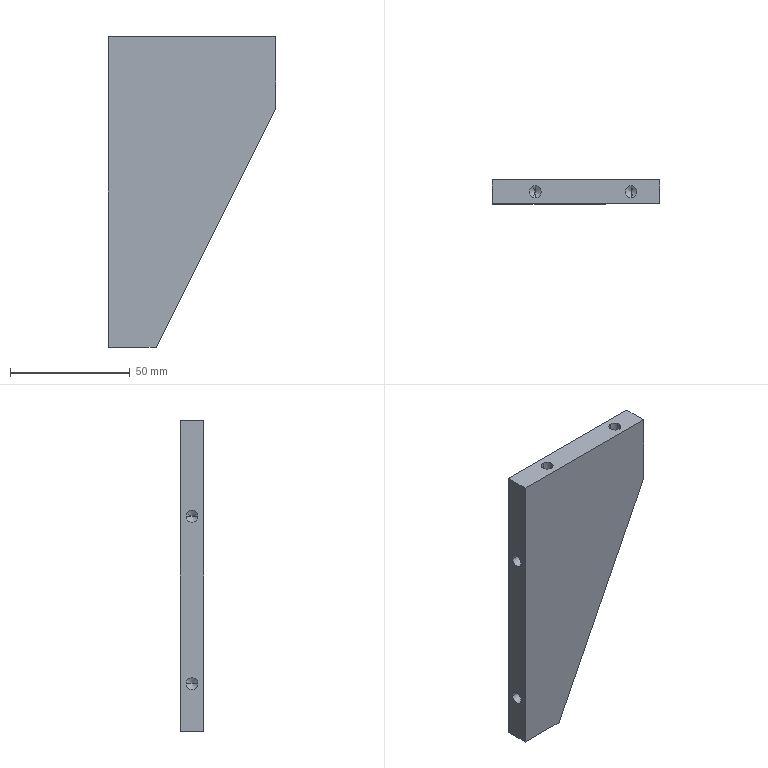Component | SolidWorks | 01-06MarkingMachineMountingReinforcementPlate-1 | 1 solid | 23 faces | box 70 x 10 x 130 mm | volume 64783 mm3 | cylinder 8 | cone 8 | plane 7 | commonest cylinder face diameters 5 x8 | material A3 Steel
build123d program:
from build123d import *

# Parameters (mm, degrees)
BOSS_EXTRUDE1_DEPTH   = 5
M6_TAPPED_HOLE1_D     = 5
M6_TAPPED_HOLE1_DEPTH = 15
M6_TAPPED_HOLE1_TIP   = 1.502
M6_TAPPED_HOLE2_D     = 5
M6_TAPPED_HOLE2_DEPTH = 15
M6_TAPPED_HOLE2_TIP   = 1.502


with BuildPart() as part:
    # Sketch1 → Boss-Extrude1 (new, symmetric)
    with BuildSketch(Plane.XY):
        Polygon((0, 130), (0, 0), (-70, 0), (-70, 30), (-20, 130), align=None)
    extrude(amount=BOSS_EXTRUDE1_DEPTH, both=True)

    # M6 Tapped Hole1
    with Locations(Plane(origin=(0, 110, 0), x_dir=(0, 0, 1), z_dir=(1, 0, 0))):
        with Locations((0, 0), (0, 70)):
            Hole(M6_TAPPED_HOLE1_D / 2, depth=M6_TAPPED_HOLE1_DEPTH)
            with Locations((0, 0, -(M6_TAPPED_HOLE1_DEPTH + M6_TAPPED_HOLE1_TIP / 2))):  # 118° drill point
                Cone(0, M6_TAPPED_HOLE1_D / 2, M6_TAPPED_HOLE1_TIP, mode=Mode.SUBTRACT)

    # M6 Tapped Hole2
    with Locations(Plane(origin=(-18, 0, 0), x_dir=(-1, 0, 0), z_dir=(0, -1, 0))):
        with Locations((0, 0), (40, 0)):
            Hole(M6_TAPPED_HOLE2_D / 2, depth=M6_TAPPED_HOLE2_DEPTH)
            with Locations((0, 0, -(M6_TAPPED_HOLE2_DEPTH + M6_TAPPED_HOLE2_TIP / 2))):  # 118° drill point
                Cone(0, M6_TAPPED_HOLE2_D / 2, M6_TAPPED_HOLE2_TIP, mode=Mode.SUBTRACT)


solid = part.part

# Placed as in the assembly
solid = solid.moved(Location((-46.91, 2.41, 85), (90, 0, -180)))
STEP:
#1=CARTESIAN_POINT('',(-1.138,-0.003525,2.756));
#2=VERTEX_POINT('',#1);
#3=CARTESIAN_POINT('',(-1.138,0.1933,2.756));
#4=VERTEX_POINT('',#3);
#5=CARTESIAN_POINT('',(-1.138,0.0949,2.756));
#6=DIRECTION('',(0.,0.,1.));
#7=DIRECTION('',(0.,1.,0.));
#8=AXIS2_PLACEMENT_3D('',#5,#6,#7);
#9=CIRCLE('',#8,0.09843);
#10=EDGE_CURVE('',#2,#4,#9,.T.);
#11=ORIENTED_EDGE('',*,*,#10,.F.);
#12=CARTESIAN_POINT('',(-1.138,-0.003525,3.346));
#13=VERTEX_POINT('',#12);
#14=CARTESIAN_POINT('',(-1.138,-0.003525,3.346));
#15=DIRECTION('',(0.,0.,1.));
#16=VECTOR('',#15,39.37);
#17=LINE('',#14,#16);
#18=EDGE_CURVE('',#2,#13,#17,.T.);
#19=ORIENTED_EDGE('',*,*,#18,.T.);
#20=CARTESIAN_POINT('',(-1.138,0.1933,3.346));
#21=VERTEX_POINT('',#20);
#22=CARTESIAN_POINT('',(-1.138,0.0949,3.346));
#23=DIRECTION('',(0.,0.,1.));
#24=DIRECTION('',(0.,1.,0.));
#25=AXIS2_PLACEMENT_3D('',#22,#23,#24);
#26=CIRCLE('',#25,0.09843);
#27=EDGE_CURVE('',#13,#21,#26,.T.);
#28=ORIENTED_EDGE('',*,*,#27,.T.);
#29=CARTESIAN_POINT('',(-1.138,0.1933,3.346));
#30=DIRECTION('',(0.,0.,1.));
#31=VECTOR('',#30,39.37);
#32=LINE('',#29,#31);
#33=EDGE_CURVE('',#4,#21,#32,.T.);
#34=ORIENTED_EDGE('',*,*,#33,.F.);
#35=EDGE_LOOP('',(#11,#19,#28,#34));
#36=FACE_OUTER_BOUND('',#35,.T.);
#37=CARTESIAN_POINT('',(-1.138,0.0949,3.346));
#38=DIRECTION('',(0.,0.,1.));
#39=DIRECTION('',(0.,1.,0.));
#40=AXIS2_PLACEMENT_3D('',#37,#38,#39);
#41=CYLINDRICAL_SURFACE('',#40,0.09843);
#42=ADVANCED_FACE('',(#36),#41,.F.);
#43=CARTESIAN_POINT('',(-1.138,0.0949,2.697));
#44=VERTEX_POINT('',#43);
#45=CARTESIAN_POINT('',(-1.138,0.1933,2.756));
#46=DIRECTION('',(0.,0.8572,0.515));
#47=VECTOR('',#46,39.37);
#48=LINE('',#45,#47);
#49=EDGE_CURVE('',#44,#4,#48,.T.);
#50=ORIENTED_EDGE('',*,*,#49,.F.);
#51=CARTESIAN_POINT('',(-1.138,-0.003525,2.756));
#52=DIRECTION('',(0.,-0.8572,0.515));
#53=VECTOR('',#52,39.37);
#54=LINE('',#51,#53);
#55=EDGE_CURVE('',#44,#2,#54,.T.);
#56=ORIENTED_EDGE('',*,*,#55,.T.);
#57=ORIENTED_EDGE('',*,*,#10,.T.);
#58=EDGE_LOOP('',(#50,#56,#57));
#59=FACE_OUTER_BOUND('',#58,.T.);
#60=CARTESIAN_POINT('',(-1.138,0.0949,2.756));
#61=DIRECTION('',(0.,0.,1.));
#62=DIRECTION('',(0.,1.,0.));
#63=AXIS2_PLACEMENT_3D('',#60,#61,#62);
#64=CONICAL_SURFACE('',#63,0.09843,1.03);
#65=ADVANCED_FACE('',(#59),#64,.F.);
#66=CARTESIAN_POINT('',(0.4366,-0.003525,2.756));
#67=VERTEX_POINT('',#66);
#68=CARTESIAN_POINT('',(0.4366,0.1933,2.756));
#69=VERTEX_POINT('',#68);
#70=CARTESIAN_POINT('',(0.4366,0.0949,2.756));
#71=DIRECTION('',(0.,0.,1.));
#72=DIRECTION('',(0.,1.,0.));
#73=AXIS2_PLACEMENT_3D('',#70,#71,#72);
#74=CIRCLE('',#73,0.09843);
#75=EDGE_CURVE('',#67,#69,#74,.T.);
#76=ORIENTED_EDGE('',*,*,#75,.F.);
#77=CARTESIAN_POINT('',(0.4366,-0.003525,3.346));
#78=VERTEX_POINT('',#77);
#79=CARTESIAN_POINT('',(0.4366,-0.003525,3.346));
#80=DIRECTION('',(0.,0.,1.));
#81=VECTOR('',#80,39.37);
#82=LINE('',#79,#81);
#83=EDGE_CURVE('',#67,#78,#82,.T.);
#84=ORIENTED_EDGE('',*,*,#83,.T.);
#85=CARTESIAN_POINT('',(0.4366,0.1933,3.346));
#86=VERTEX_POINT('',#85);
#87=CARTESIAN_POINT('',(0.4366,0.0949,3.346));
#88=DIRECTION('',(0.,0.,1.));
#89=DIRECTION('',(0.,1.,0.));
#90=AXIS2_PLACEMENT_3D('',#87,#88,#89);
#91=CIRCLE('',#90,0.09843);
#92=EDGE_CURVE('',#78,#86,#91,.T.);
#93=ORIENTED_EDGE('',*,*,#92,.T.);
#94=CARTESIAN_POINT('',(0.4366,0.1933,3.346));
#95=DIRECTION('',(0.,0.,1.));
#96=VECTOR('',#95,39.37);
#97=LINE('',#94,#96);
#98=EDGE_CURVE('',#69,#86,#97,.T.);
#99=ORIENTED_EDGE('',*,*,#98,.F.);
#100=EDGE_LOOP('',(#76,#84,#93,#99));
#101=FACE_OUTER_BOUND('',#100,.T.);
#102=CARTESIAN_POINT('',(0.4366,0.0949,3.346));
#103=DIRECTION('',(0.,0.,1.));
#104=DIRECTION('',(0.,1.,0.));
#105=AXIS2_PLACEMENT_3D('',#102,#103,#104);
#106=CYLINDRICAL_SURFACE('',#105,0.09843);
#107=ADVANCED_FACE('',(#101),#106,.F.);
#108=CARTESIAN_POINT('',(0.4366,0.0949,2.697));
#109=VERTEX_POINT('',#108);
#110=CARTESIAN_POINT('',(0.4366,0.1933,2.756));
#111=DIRECTION('',(0.,0.8572,0.515));
#112=VECTOR('',#111,39.37);
#113=LINE('',#110,#112);
#114=EDGE_CURVE('',#109,#69,#113,.T.);
#115=ORIENTED_EDGE('',*,*,#114,.F.);
#116=CARTESIAN_POINT('',(0.4366,-0.003525,2.756));
#117=DIRECTION('',(0.,-0.8572,0.515));
#118=VECTOR('',#117,39.37);
#119=LINE('',#116,#118);
#120=EDGE_CURVE('',#109,#67,#119,.T.);
#121=ORIENTED_EDGE('',*,*,#120,.T.);
#122=ORIENTED_EDGE('',*,*,#75,.T.);
#123=EDGE_LOOP('',(#115,#121,#122));
#124=FACE_OUTER_BOUND('',#123,.T.);
#125=CARTESIAN_POINT('',(0.4366,0.0949,2.756));
#126=DIRECTION('',(0.,0.,1.));
#127=DIRECTION('',(0.,1.,0.));
#128=AXIS2_PLACEMENT_3D('',#125,#126,#127);
#129=CONICAL_SURFACE('',#128,0.09843,1.03);
#130=ADVANCED_FACE('',(#124),#129,.F.);
#131=CARTESIAN_POINT('',(-1.256,-0.003525,-0.9843));
#132=VERTEX_POINT('',#131);
#133=CARTESIAN_POINT('',(-1.256,0.1933,-0.9843));
#134=VERTEX_POINT('',#133);
#135=CARTESIAN_POINT('',(-1.256,0.0949,-0.9843));
#136=DIRECTION('',(-1.,-0.,0.));
#137=DIRECTION('',(0.,1.,0.));
#138=AXIS2_PLACEMENT_3D('',#135,#136,#137);
#139=CIRCLE('',#138,0.09843);
#140=EDGE_CURVE('',#132,#134,#139,.T.);
#141=ORIENTED_EDGE('',*,*,#140,.F.);
#142=CARTESIAN_POINT('',(-1.847,-0.003525,-0.9843));
#143=VERTEX_POINT('',#142);
#144=CARTESIAN_POINT('',(-1.847,-0.003525,-0.9843));
#145=DIRECTION('',(-1.,-0.,0.));
#146=VECTOR('',#145,39.37);
#147=LINE('',#144,#146);
#148=EDGE_CURVE('',#132,#143,#147,.T.);
#149=ORIENTED_EDGE('',*,*,#148,.T.);
#150=CARTESIAN_POINT('',(-1.847,0.1933,-0.9843));
#151=VERTEX_POINT('',#150);
#152=CARTESIAN_POINT('',(-1.847,0.0949,-0.9843));
#153=DIRECTION('',(-1.,-0.,0.));
#154=DIRECTION('',(0.,1.,0.));
#155=AXIS2_PLACEMENT_3D('',#152,#153,#154);
#156=CIRCLE('',#155,0.09843);
#157=EDGE_CURVE('',#143,#151,#156,.T.);
#158=ORIENTED_EDGE('',*,*,#157,.T.);
#159=CARTESIAN_POINT('',(-1.847,0.1933,-0.9843));
#160=DIRECTION('',(-1.,-0.,0.));
#161=VECTOR('',#160,39.37);
#162=LINE('',#159,#161);
#163=EDGE_CURVE('',#134,#151,#162,.T.);
#164=ORIENTED_EDGE('',*,*,#163,.F.);
#165=EDGE_LOOP('',(#141,#149,#158,#164));
#166=FACE_OUTER_BOUND('',#165,.T.);
#167=CARTESIAN_POINT('',(-1.847,0.0949,-0.9843));
#168=DIRECTION('',(-1.,-0.,0.));
#169=DIRECTION('',(0.,1.,0.));
#170=AXIS2_PLACEMENT_3D('',#167,#168,#169);
#171=CYLINDRICAL_SURFACE('',#170,0.09843);
#172=ADVANCED_FACE('',(#166),#171,.F.);
#173=CARTESIAN_POINT('',(-1.197,0.0949,-0.9843));
#174=VERTEX_POINT('',#173);
#175=CARTESIAN_POINT('',(-1.256,0.1933,-0.9843));
#176=DIRECTION('',(-0.515,0.8572,0.));
#177=VECTOR('',#176,39.37);
#178=LINE('',#175,#177);
#179=EDGE_CURVE('',#174,#134,#178,.T.);
#180=ORIENTED_EDGE('',*,*,#179,.F.);
#181=CARTESIAN_POINT('',(-1.256,-0.003525,-0.9843));
#182=DIRECTION('',(-0.515,-0.8572,0.));
#183=VECTOR('',#182,39.37);
#184=LINE('',#181,#183);
#185=EDGE_CURVE('',#174,#132,#184,.T.);
#186=ORIENTED_EDGE('',*,*,#185,.T.);
#187=ORIENTED_EDGE('',*,*,#140,.T.);
#188=EDGE_LOOP('',(#180,#186,#187));
#189=FACE_OUTER_BOUND('',#188,.T.);
#190=CARTESIAN_POINT('',(-1.256,0.0949,-0.9843));
#191=DIRECTION('',(-1.,-0.,0.));
#192=DIRECTION('',(0.,1.,0.));
#193=AXIS2_PLACEMENT_3D('',#190,#191,#192);
#194=CONICAL_SURFACE('',#193,0.09843,1.03);
#195=ADVANCED_FACE('',(#189),#194,.F.);
#196=CARTESIAN_POINT('',(-1.256,-0.003525,1.772));
#197=VERTEX_POINT('',#196);
#198=CARTESIAN_POINT('',(-1.256,0.1933,1.772));
#199=VERTEX_POINT('',#198);
#200=CARTESIAN_POINT('',(-1.256,0.0949,1.772));
#201=DIRECTION('',(-1.,-0.,0.));
#202=DIRECTION('',(0.,1.,0.));
#203=AXIS2_PLACEMENT_3D('',#200,#201,#202);
#204=CIRCLE('',#203,0.09843);
#205=EDGE_CURVE('',#197,#199,#204,.T.);
#206=ORIENTED_EDGE('',*,*,#205,.F.);
#207=CARTESIAN_POINT('',(-1.847,-0.003525,1.772));
#208=VERTEX_POINT('',#207);
#209=CARTESIAN_POINT('',(-1.847,-0.003525,1.772));
#210=DIRECTION('',(-1.,-0.,0.));
#211=VECTOR('',#210,39.37);
#212=LINE('',#209,#211);
#213=EDGE_CURVE('',#197,#208,#212,.T.);
#214=ORIENTED_EDGE('',*,*,#213,.T.);
#215=CARTESIAN_POINT('',(-1.847,0.1933,1.772));
#216=VERTEX_POINT('',#215);
#217=CARTESIAN_POINT('',(-1.847,0.0949,1.772));
#218=DIRECTION('',(-1.,-0.,0.));
#219=DIRECTION('',(0.,1.,0.));
#220=AXIS2_PLACEMENT_3D('',#217,#218,#219);
#221=CIRCLE('',#220,0.09843);
#222=EDGE_CURVE('',#208,#216,#221,.T.);
#223=ORIENTED_EDGE('',*,*,#222,.T.);
#224=CARTESIAN_POINT('',(-1.847,0.1933,1.772));
#225=DIRECTION('',(-1.,-0.,0.));
#226=VECTOR('',#225,39.37);
#227=LINE('',#224,#226);
#228=EDGE_CURVE('',#199,#216,#227,.T.);
#229=ORIENTED_EDGE('',*,*,#228,.F.);
#230=EDGE_LOOP('',(#206,#214,#223,#229));
#231=FACE_OUTER_BOUND('',#230,.T.);
#232=CARTESIAN_POINT('',(-1.847,0.0949,1.772));
#233=DIRECTION('',(-1.,-0.,0.));
#234=DIRECTION('',(0.,1.,0.));
#235=AXIS2_PLACEMENT_3D('',#232,#233,#234);
#236=CYLINDRICAL_SURFACE('',#235,0.09843);
#237=ADVANCED_FACE('',(#231),#236,.F.);
#238=CARTESIAN_POINT('',(-1.197,0.0949,1.772));
#239=VERTEX_POINT('',#238);
#240=CARTESIAN_POINT('',(-1.256,0.1933,1.772));
#241=DIRECTION('',(-0.515,0.8572,0.));
#242=VECTOR('',#241,39.37);
#243=LINE('',#240,#242);
#244=EDGE_CURVE('',#239,#199,#243,.T.);
#245=ORIENTED_EDGE('',*,*,#244,.F.);
#246=CARTESIAN_POINT('',(-1.256,-0.003525,1.772));
#247=DIRECTION('',(-0.515,-0.8572,0.));
#248=VECTOR('',#247,39.37);
#249=LINE('',#246,#248);
#250=EDGE_CURVE('',#239,#197,#249,.T.);
#251=ORIENTED_EDGE('',*,*,#250,.T.);
#252=ORIENTED_EDGE('',*,*,#205,.T.);
#253=EDGE_LOOP('',(#245,#251,#252));
#254=FACE_OUTER_BOUND('',#253,.T.);
#255=CARTESIAN_POINT('',(-1.256,0.0949,1.772));
#256=DIRECTION('',(-1.,-0.,0.));
#257=DIRECTION('',(0.,1.,0.));
#258=AXIS2_PLACEMENT_3D('',#255,#256,#257);
#259=CONICAL_SURFACE('',#258,0.09843,1.03);
#260=ADVANCED_FACE('',(#254),#259,.F.);
#261=CARTESIAN_POINT('',(-1.847,0.2918,-1.772));
#262=VERTEX_POINT('',#261);
#263=CARTESIAN_POINT('',(-1.059,0.2918,-1.772));
#264=VERTEX_POINT('',#263);
#265=CARTESIAN_POINT('',(-1.059,0.2918,-1.772));
#266=DIRECTION('',(1.,0.,-0.));
#267=VECTOR('',#266,39.37);
#268=LINE('',#265,#267);
#269=EDGE_CURVE('',#262,#264,#268,.T.);
#270=ORIENTED_EDGE('',*,*,#269,.T.);
#271=CARTESIAN_POINT('',(-1.059,-0.102,-1.772));
#272=VERTEX_POINT('',#271);
#273=CARTESIAN_POINT('',(-1.059,-0.102,-1.772));
#274=DIRECTION('',(-0.,1.,0.));
#275=VECTOR('',#274,39.37);
#276=LINE('',#273,#275);
#277=EDGE_CURVE('',#272,#264,#276,.T.);
#278=ORIENTED_EDGE('',*,*,#277,.F.);
#279=CARTESIAN_POINT('',(-1.847,-0.102,-1.772));
#280=VERTEX_POINT('',#279);
#281=CARTESIAN_POINT('',(-1.059,-0.102,-1.772));
#282=DIRECTION('',(1.,0.,-0.));
#283=VECTOR('',#282,39.37);
#284=LINE('',#281,#283);
#285=EDGE_CURVE('',#280,#272,#284,.T.);
#286=ORIENTED_EDGE('',*,*,#285,.F.);
#287=CARTESIAN_POINT('',(-1.847,-0.102,-1.772));
#288=DIRECTION('',(-0.,1.,0.));
#289=VECTOR('',#288,39.37);
#290=LINE('',#287,#289);
#291=EDGE_CURVE('',#280,#262,#290,.T.);
#292=ORIENTED_EDGE('',*,*,#291,.T.);
#293=EDGE_LOOP('',(#270,#278,#286,#292));
#294=FACE_OUTER_BOUND('',#293,.T.);
#295=CARTESIAN_POINT('',(-1.059,-0.102,-1.772));
#296=DIRECTION('',(0.,-0.,1.));
#297=DIRECTION('',(-0.,1.,0.));
#298=AXIS2_PLACEMENT_3D('',#295,#296,#297);
#299=PLANE('',#298);
#300=ADVANCED_FACE('',(#294),#299,.F.);
#301=CARTESIAN_POINT('',(0.909,0.2918,2.165));
#302=VERTEX_POINT('',#301);
#303=CARTESIAN_POINT('',(0.909,0.2918,2.165));
#304=DIRECTION('',(0.4472,0.,0.8944));
#305=VECTOR('',#304,39.37);
#306=LINE('',#303,#305);
#307=EDGE_CURVE('',#264,#302,#306,.T.);
#308=ORIENTED_EDGE('',*,*,#307,.T.);
#309=CARTESIAN_POINT('',(0.909,-0.102,2.165));
#310=VERTEX_POINT('',#309);
#311=CARTESIAN_POINT('',(0.909,-0.102,2.165));
#312=DIRECTION('',(-0.,1.,0.));
#313=VECTOR('',#312,39.37);
#314=LINE('',#311,#313);
#315=EDGE_CURVE('',#310,#302,#314,.T.);
#316=ORIENTED_EDGE('',*,*,#315,.F.);
#317=CARTESIAN_POINT('',(0.909,-0.102,2.165));
#318=DIRECTION('',(0.4472,0.,0.8944));
#319=VECTOR('',#318,39.37);
#320=LINE('',#317,#319);
#321=EDGE_CURVE('',#272,#310,#320,.T.);
#322=ORIENTED_EDGE('',*,*,#321,.F.);
#323=ORIENTED_EDGE('',*,*,#277,.T.);
#324=EDGE_LOOP('',(#308,#316,#322,#323));
#325=FACE_OUTER_BOUND('',#324,.T.);
#326=CARTESIAN_POINT('',(0.909,-0.102,2.165));
#327=DIRECTION('',(-0.8944,-0.,0.4472));
#328=DIRECTION('',(-0.4472,-0.,-0.8944));
#329=AXIS2_PLACEMENT_3D('',#326,#327,#328);
#330=PLANE('',#329);
#331=ADVANCED_FACE('',(#325),#330,.F.);
#332=CARTESIAN_POINT('',(0.909,0.2918,3.346));
#333=VERTEX_POINT('',#332);
#334=CARTESIAN_POINT('',(0.909,0.2918,3.346));
#335=DIRECTION('',(0.,0.,1.));
#336=VECTOR('',#335,39.37);
#337=LINE('',#334,#336);
#338=EDGE_CURVE('',#302,#333,#337,.T.);
#339=ORIENTED_EDGE('',*,*,#338,.T.);
#340=CARTESIAN_POINT('',(0.909,-0.102,3.346));
#341=VERTEX_POINT('',#340);
#342=CARTESIAN_POINT('',(0.909,-0.102,3.346));
#343=DIRECTION('',(-0.,1.,0.));
#344=VECTOR('',#343,39.37);
#345=LINE('',#342,#344);
#346=EDGE_CURVE('',#341,#333,#345,.T.);
#347=ORIENTED_EDGE('',*,*,#346,.F.);
#348=CARTESIAN_POINT('',(0.909,-0.102,3.346));
#349=DIRECTION('',(0.,0.,1.));
#350=VECTOR('',#349,39.37);
#351=LINE('',#348,#350);
#352=EDGE_CURVE('',#310,#341,#351,.T.);
#353=ORIENTED_EDGE('',*,*,#352,.F.);
#354=ORIENTED_EDGE('',*,*,#315,.T.);
#355=EDGE_LOOP('',(#339,#347,#353,#354));
#356=FACE_OUTER_BOUND('',#355,.T.);
#357=CARTESIAN_POINT('',(0.909,-0.102,3.346));
#358=DIRECTION('',(-1.,-0.,0.));
#359=DIRECTION('',(-0.,1.,0.));
#360=AXIS2_PLACEMENT_3D('',#357,#358,#359);
#361=PLANE('',#360);
#362=ADVANCED_FACE('',(#356),#361,.F.);
#363=CARTESIAN_POINT('',(-1.138,0.0949,3.346));
#364=DIRECTION('',(0.,0.,1.));
#365=DIRECTION('',(0.,1.,0.));
#366=AXIS2_PLACEMENT_3D('',#363,#364,#365);
#367=CIRCLE('',#366,0.09843);
#368=EDGE_CURVE('',#21,#13,#367,.T.);
#369=ORIENTED_EDGE('',*,*,#368,.F.);
#370=ORIENTED_EDGE('',*,*,#27,.F.);
#371=EDGE_LOOP('',(#369,#370));
#372=FACE_BOUND('',#371,.T.);
#373=CARTESIAN_POINT('',(0.4366,0.0949,3.346));
#374=DIRECTION('',(0.,0.,1.));
#375=DIRECTION('',(0.,1.,0.));
#376=AXIS2_PLACEMENT_3D('',#373,#374,#375);
#377=CIRCLE('',#376,0.09843);
#378=EDGE_CURVE('',#86,#78,#377,.T.);
#379=ORIENTED_EDGE('',*,*,#378,.F.);
#380=ORIENTED_EDGE('',*,*,#92,.F.);
#381=EDGE_LOOP('',(#379,#380));
#382=FACE_BOUND('',#381,.T.);
#383=CARTESIAN_POINT('',(-1.847,0.2918,3.346));
#384=VERTEX_POINT('',#383);
#385=CARTESIAN_POINT('',(-1.847,0.2918,3.346));
#386=DIRECTION('',(-1.,-0.,0.));
#387=VECTOR('',#386,39.37);
#388=LINE('',#385,#387);
#389=EDGE_CURVE('',#333,#384,#388,.T.);
#390=ORIENTED_EDGE('',*,*,#389,.T.);
#391=CARTESIAN_POINT('',(-1.847,-0.102,3.346));
#392=VERTEX_POINT('',#391);
#393=CARTESIAN_POINT('',(-1.847,-0.102,3.346));
#394=DIRECTION('',(-0.,1.,0.));
#395=VECTOR('',#394,39.37);
#396=LINE('',#393,#395);
#397=EDGE_CURVE('',#392,#384,#396,.T.);
#398=ORIENTED_EDGE('',*,*,#397,.F.);
#399=CARTESIAN_POINT('',(-1.847,-0.102,3.346));
#400=DIRECTION('',(-1.,-0.,0.));
#401=VECTOR('',#400,39.37);
#402=LINE('',#399,#401);
#403=EDGE_CURVE('',#341,#392,#402,.T.);
#404=ORIENTED_EDGE('',*,*,#403,.F.);
#405=ORIENTED_EDGE('',*,*,#346,.T.);
#406=EDGE_LOOP('',(#390,#398,#404,#405));
#407=FACE_OUTER_BOUND('',#406,.T.);
#408=CARTESIAN_POINT('',(-1.847,-0.102,3.346));
#409=DIRECTION('',(-0.,0.,-1.));
#410=DIRECTION('',(1.,0.,-0.));
#411=AXIS2_PLACEMENT_3D('',#408,#409,#410);
#412=PLANE('',#411);
#413=ADVANCED_FACE('',(#372,#382,#407),#412,.F.);
#414=CARTESIAN_POINT('',(-1.847,0.0949,-0.9843));
#415=DIRECTION('',(-1.,-0.,0.));
#416=DIRECTION('',(0.,1.,0.));
#417=AXIS2_PLACEMENT_3D('',#414,#415,#416);
#418=CIRCLE('',#417,0.09843);
#419=EDGE_CURVE('',#151,#143,#418,.T.);
#420=ORIENTED_EDGE('',*,*,#419,.F.);
#421=ORIENTED_EDGE('',*,*,#157,.F.);
#422=EDGE_LOOP('',(#420,#421));
#423=FACE_BOUND('',#422,.T.);
#424=CARTESIAN_POINT('',(-1.847,0.0949,1.772));
#425=DIRECTION('',(-1.,-0.,0.));
#426=DIRECTION('',(0.,1.,0.));
#427=AXIS2_PLACEMENT_3D('',#424,#425,#426);
#428=CIRCLE('',#427,0.09843);
#429=EDGE_CURVE('',#216,#208,#428,.T.);
#430=ORIENTED_EDGE('',*,*,#429,.F.);
#431=ORIENTED_EDGE('',*,*,#222,.F.);
#432=EDGE_LOOP('',(#430,#431));
#433=FACE_BOUND('',#432,.T.);
#434=CARTESIAN_POINT('',(-1.847,0.2918,-1.772));
#435=DIRECTION('',(-0.,-0.,-1.));
#436=VECTOR('',#435,39.37);
#437=LINE('',#434,#436);
#438=EDGE_CURVE('',#384,#262,#437,.T.);
#439=ORIENTED_EDGE('',*,*,#438,.T.);
#440=ORIENTED_EDGE('',*,*,#291,.F.);
#441=CARTESIAN_POINT('',(-1.847,-0.102,-1.772));
#442=DIRECTION('',(-0.,-0.,-1.));
#443=VECTOR('',#442,39.37);
#444=LINE('',#441,#443);
#445=EDGE_CURVE('',#392,#280,#444,.T.);
#446=ORIENTED_EDGE('',*,*,#445,.F.);
#447=ORIENTED_EDGE('',*,*,#397,.T.);
#448=EDGE_LOOP('',(#439,#440,#446,#447));
#449=FACE_OUTER_BOUND('',#448,.T.);
#450=CARTESIAN_POINT('',(-1.847,-0.102,-1.772));
#451=DIRECTION('',(1.,0.,-0.));
#452=DIRECTION('',(0.,-1.,-0.));
#453=AXIS2_PLACEMENT_3D('',#450,#451,#452);
#454=PLANE('',#453);
#455=ADVANCED_FACE('',(#423,#433,#449),#454,.F.);
#456=ORIENTED_EDGE('',*,*,#285,.T.);
#457=ORIENTED_EDGE('',*,*,#321,.T.);
#458=ORIENTED_EDGE('',*,*,#352,.T.);
#459=ORIENTED_EDGE('',*,*,#403,.T.);
#460=ORIENTED_EDGE('',*,*,#445,.T.);
#461=EDGE_LOOP('',(#456,#457,#458,#459,#460));
#462=FACE_OUTER_BOUND('',#461,.T.);
#463=CARTESIAN_POINT('',(-1.847,-0.102,3.346));
#464=DIRECTION('',(-0.,1.,0.));
#465=DIRECTION('',(1.,0.,-0.));
#466=AXIS2_PLACEMENT_3D('',#463,#464,#465);
#467=PLANE('',#466);
#468=ADVANCED_FACE('',(#462),#467,.F.);
#469=ORIENTED_EDGE('',*,*,#269,.F.);
#470=ORIENTED_EDGE('',*,*,#438,.F.);
#471=ORIENTED_EDGE('',*,*,#389,.F.);
#472=ORIENTED_EDGE('',*,*,#338,.F.);
#473=ORIENTED_EDGE('',*,*,#307,.F.);
#474=EDGE_LOOP('',(#469,#470,#471,#472,#473));
#475=FACE_OUTER_BOUND('',#474,.T.);
#476=CARTESIAN_POINT('',(-1.847,0.2918,3.346));
#477=DIRECTION('',(-0.,1.,0.));
#478=DIRECTION('',(1.,0.,-0.));
#479=AXIS2_PLACEMENT_3D('',#476,#477,#478);
#480=PLANE('',#479);
#481=ADVANCED_FACE('',(#475),#480,.T.);
#482=ORIENTED_EDGE('',*,*,#250,.F.);
#483=ORIENTED_EDGE('',*,*,#244,.T.);
#484=CARTESIAN_POINT('',(-1.256,0.0949,1.772));
#485=DIRECTION('',(-1.,-0.,0.));
#486=DIRECTION('',(0.,1.,0.));
#487=AXIS2_PLACEMENT_3D('',#484,#485,#486);
#488=CIRCLE('',#487,0.09843);
#489=EDGE_CURVE('',#199,#197,#488,.T.);
#490=ORIENTED_EDGE('',*,*,#489,.T.);
#491=EDGE_LOOP('',(#482,#483,#490));
#492=FACE_OUTER_BOUND('',#491,.T.);
#493=CARTESIAN_POINT('',(-1.256,0.0949,1.772));
#494=DIRECTION('',(-1.,-0.,0.));
#495=DIRECTION('',(0.,1.,0.));
#496=AXIS2_PLACEMENT_3D('',#493,#494,#495);
#497=CONICAL_SURFACE('',#496,0.09843,1.03);
#498=ADVANCED_FACE('',(#492),#497,.F.);
#499=ORIENTED_EDGE('',*,*,#213,.F.);
#500=ORIENTED_EDGE('',*,*,#489,.F.);
#501=ORIENTED_EDGE('',*,*,#228,.T.);
#502=ORIENTED_EDGE('',*,*,#429,.T.);
#503=EDGE_LOOP('',(#499,#500,#501,#502));
#504=FACE_OUTER_BOUND('',#503,.T.);
#505=CARTESIAN_POINT('',(-1.847,0.0949,1.772));
#506=DIRECTION('',(-1.,-0.,0.));
#507=DIRECTION('',(0.,1.,0.));
#508=AXIS2_PLACEMENT_3D('',#505,#506,#507);
#509=CYLINDRICAL_SURFACE('',#508,0.09843);
#510=ADVANCED_FACE('',(#504),#509,.F.);
#511=ORIENTED_EDGE('',*,*,#185,.F.);
#512=ORIENTED_EDGE('',*,*,#179,.T.);
#513=CARTESIAN_POINT('',(-1.256,0.0949,-0.9843));
#514=DIRECTION('',(-1.,-0.,0.));
#515=DIRECTION('',(0.,1.,0.));
#516=AXIS2_PLACEMENT_3D('',#513,#514,#515);
#517=CIRCLE('',#516,0.09843);
#518=EDGE_CURVE('',#134,#132,#517,.T.);
#519=ORIENTED_EDGE('',*,*,#518,.T.);
#520=EDGE_LOOP('',(#511,#512,#519));
#521=FACE_OUTER_BOUND('',#520,.T.);
#522=CARTESIAN_POINT('',(-1.256,0.0949,-0.9843));
#523=DIRECTION('',(-1.,-0.,0.));
#524=DIRECTION('',(0.,1.,0.));
#525=AXIS2_PLACEMENT_3D('',#522,#523,#524);
#526=CONICAL_SURFACE('',#525,0.09843,1.03);
#527=ADVANCED_FACE('',(#521),#526,.F.);
#528=ORIENTED_EDGE('',*,*,#148,.F.);
#529=ORIENTED_EDGE('',*,*,#518,.F.);
#530=ORIENTED_EDGE('',*,*,#163,.T.);
#531=ORIENTED_EDGE('',*,*,#419,.T.);
#532=EDGE_LOOP('',(#528,#529,#530,#531));
#533=FACE_OUTER_BOUND('',#532,.T.);
#534=CARTESIAN_POINT('',(-1.847,0.0949,-0.9843));
#535=DIRECTION('',(-1.,-0.,0.));
#536=DIRECTION('',(0.,1.,0.));
#537=AXIS2_PLACEMENT_3D('',#534,#535,#536);
#538=CYLINDRICAL_SURFACE('',#537,0.09843);
#539=ADVANCED_FACE('',(#533),#538,.F.);
#540=ORIENTED_EDGE('',*,*,#120,.F.);
#541=ORIENTED_EDGE('',*,*,#114,.T.);
#542=CARTESIAN_POINT('',(0.4366,0.0949,2.756));
#543=DIRECTION('',(0.,0.,1.));
#544=DIRECTION('',(0.,1.,0.));
#545=AXIS2_PLACEMENT_3D('',#542,#543,#544);
#546=CIRCLE('',#545,0.09843);
#547=EDGE_CURVE('',#69,#67,#546,.T.);
#548=ORIENTED_EDGE('',*,*,#547,.T.);
#549=EDGE_LOOP('',(#540,#541,#548));
#550=FACE_OUTER_BOUND('',#549,.T.);
#551=CARTESIAN_POINT('',(0.4366,0.0949,2.756));
#552=DIRECTION('',(0.,0.,1.));
#553=DIRECTION('',(0.,1.,0.));
#554=AXIS2_PLACEMENT_3D('',#551,#552,#553);
#555=CONICAL_SURFACE('',#554,0.09843,1.03);
#556=ADVANCED_FACE('',(#550),#555,.F.);
#557=ORIENTED_EDGE('',*,*,#83,.F.);
#558=ORIENTED_EDGE('',*,*,#547,.F.);
#559=ORIENTED_EDGE('',*,*,#98,.T.);
#560=ORIENTED_EDGE('',*,*,#378,.T.);
#561=EDGE_LOOP('',(#557,#558,#559,#560));
#562=FACE_OUTER_BOUND('',#561,.T.);
#563=CARTESIAN_POINT('',(0.4366,0.0949,3.346));
#564=DIRECTION('',(0.,0.,1.));
#565=DIRECTION('',(0.,1.,0.));
#566=AXIS2_PLACEMENT_3D('',#563,#564,#565);
#567=CYLINDRICAL_SURFACE('',#566,0.09843);
#568=ADVANCED_FACE('',(#562),#567,.F.);
#569=ORIENTED_EDGE('',*,*,#55,.F.);
#570=ORIENTED_EDGE('',*,*,#49,.T.);
#571=CARTESIAN_POINT('',(-1.138,0.0949,2.756));
#572=DIRECTION('',(0.,0.,1.));
#573=DIRECTION('',(0.,1.,0.));
#574=AXIS2_PLACEMENT_3D('',#571,#572,#573);
#575=CIRCLE('',#574,0.09843);
#576=EDGE_CURVE('',#4,#2,#575,.T.);
#577=ORIENTED_EDGE('',*,*,#576,.T.);
#578=EDGE_LOOP('',(#569,#570,#577));
#579=FACE_OUTER_BOUND('',#578,.T.);
#580=CARTESIAN_POINT('',(-1.138,0.0949,2.756));
#581=DIRECTION('',(0.,0.,1.));
#582=DIRECTION('',(0.,1.,0.));
#583=AXIS2_PLACEMENT_3D('',#580,#581,#582);
#584=CONICAL_SURFACE('',#583,0.09843,1.03);
#585=ADVANCED_FACE('',(#579),#584,.F.);
#586=ORIENTED_EDGE('',*,*,#18,.F.);
#587=ORIENTED_EDGE('',*,*,#576,.F.);
#588=ORIENTED_EDGE('',*,*,#33,.T.);
#589=ORIENTED_EDGE('',*,*,#368,.T.);
#590=EDGE_LOOP('',(#586,#587,#588,#589));
#591=FACE_OUTER_BOUND('',#590,.T.);
#592=CARTESIAN_POINT('',(-1.138,0.0949,3.346));
#593=DIRECTION('',(0.,0.,1.));
#594=DIRECTION('',(0.,1.,0.));
#595=AXIS2_PLACEMENT_3D('',#592,#593,#594);
#596=CYLINDRICAL_SURFACE('',#595,0.09843);
#597=ADVANCED_FACE('',(#591),#596,.F.);
#598=CLOSED_SHELL('',(#42,#65,#107,#130,#172,#195,#237,#260,#300,#331,#362,#413,#455,#468,#481,#498,#510,#527,#539,#556,#568,#585,#597));
#599=MANIFOLD_SOLID_BREP('',#598);
#600=CARTESIAN_POINT('',(0.,0.,0.));
#601=DIRECTION('',(0.,0.,1.));
#602=DIRECTION('',(1.,0.,0.));
#603=AXIS2_PLACEMENT_3D('',#600,#601,#602);
#604=(LENGTH_UNIT()NAMED_UNIT(*)SI_UNIT($,.METRE.));
#605=LENGTH_MEASURE_WITH_UNIT(LENGTH_MEASURE(0.0254),#604);
#606=DIMENSIONAL_EXPONENTS(1.,0.,0.,0.,0.,0.,0.);
#607=(CONVERSION_BASED_UNIT('',#605)LENGTH_UNIT()NAMED_UNIT(#606));
#608=UNCERTAINTY_MEASURE_WITH_UNIT(LENGTH_MEASURE(0.00001),#607,'','');
#609=(NAMED_UNIT(*)PLANE_ANGLE_UNIT()SI_UNIT($,.RADIAN.));
#610=(NAMED_UNIT(*)SI_UNIT($,.STERADIAN.)SOLID_ANGLE_UNIT());
#611=(GEOMETRIC_REPRESENTATION_CONTEXT(3)GLOBAL_UNCERTAINTY_ASSIGNED_CONTEXT((#608))GLOBAL_UNIT_ASSIGNED_CONTEXT((#607,#609,#610))REPRESENTATION_CONTEXT('',''));
#612=ADVANCED_BREP_SHAPE_REPRESENTATION('',(#599,#603),#611);
#613=COLOUR_RGB('',0.7922,0.8196,0.9333);
#614=FILL_AREA_STYLE_COLOUR('',#613);
#615=FILL_AREA_STYLE('',(#614));
#616=SURFACE_STYLE_FILL_AREA(#615);
#617=SURFACE_SIDE_STYLE('',(#616));
#618=SURFACE_STYLE_USAGE(.BOTH.,#617);
#619=PRESENTATION_STYLE_ASSIGNMENT((#618));
#620=STYLED_ITEM('',(#619),#599);
#621=(LENGTH_UNIT()NAMED_UNIT(*)SI_UNIT($,.METRE.));
#622=LENGTH_MEASURE_WITH_UNIT(LENGTH_MEASURE(0.0254),#621);
#623=DIMENSIONAL_EXPONENTS(1.,0.,0.,0.,0.,0.,0.);
#624=(CONVERSION_BASED_UNIT('',#622)LENGTH_UNIT()NAMED_UNIT(#623));
#625=UNCERTAINTY_MEASURE_WITH_UNIT(LENGTH_MEASURE(0.00001),#624,'','');
#626=(NAMED_UNIT(*)PLANE_ANGLE_UNIT()SI_UNIT($,.RADIAN.));
#627=(NAMED_UNIT(*)SI_UNIT($,.STERADIAN.)SOLID_ANGLE_UNIT());
#628=(GEOMETRIC_REPRESENTATION_CONTEXT(3)GLOBAL_UNCERTAINTY_ASSIGNED_CONTEXT((#625))GLOBAL_UNIT_ASSIGNED_CONTEXT((#624,#626,#627))REPRESENTATION_CONTEXT('',''));
#629=MECHANICAL_DESIGN_GEOMETRIC_PRESENTATION_REPRESENTATION('',(#620),#628);
#630=PRESENTATION_LAYER_ASSIGNMENT('','',(#620));